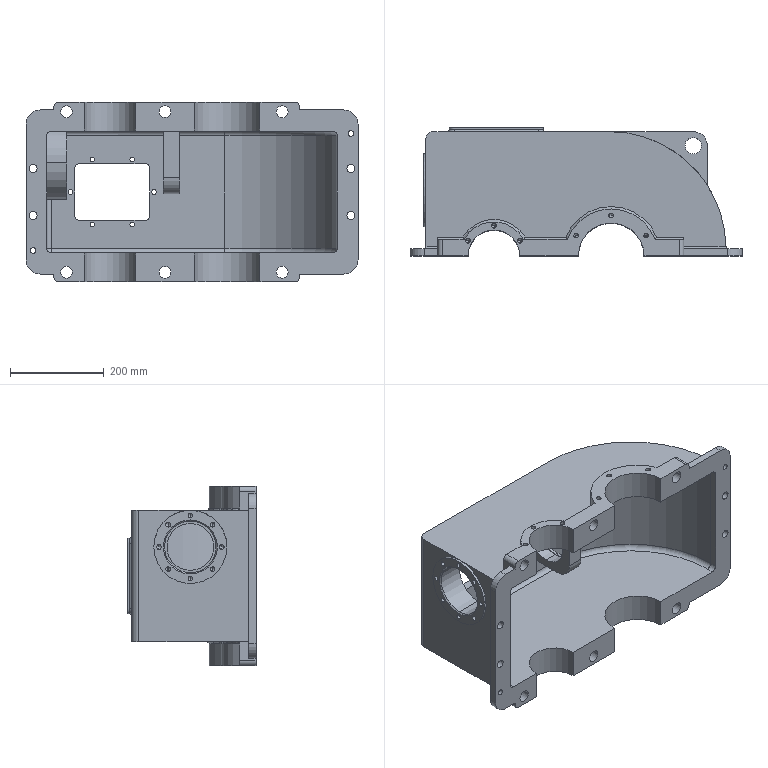Component | SolidWorks | UpperHousingAssembly-1_UpperHousing-1 | 1 solid | 248 faces | volume 8790060 mm3 | cylinder 142 | plane 53 | cone 42 | torus 10 | sphere 1 | commonest cylinder face diameters 10 x66 20 x20 25 x12 17 x8 156 x5 60 x5 12 x4 110 x4